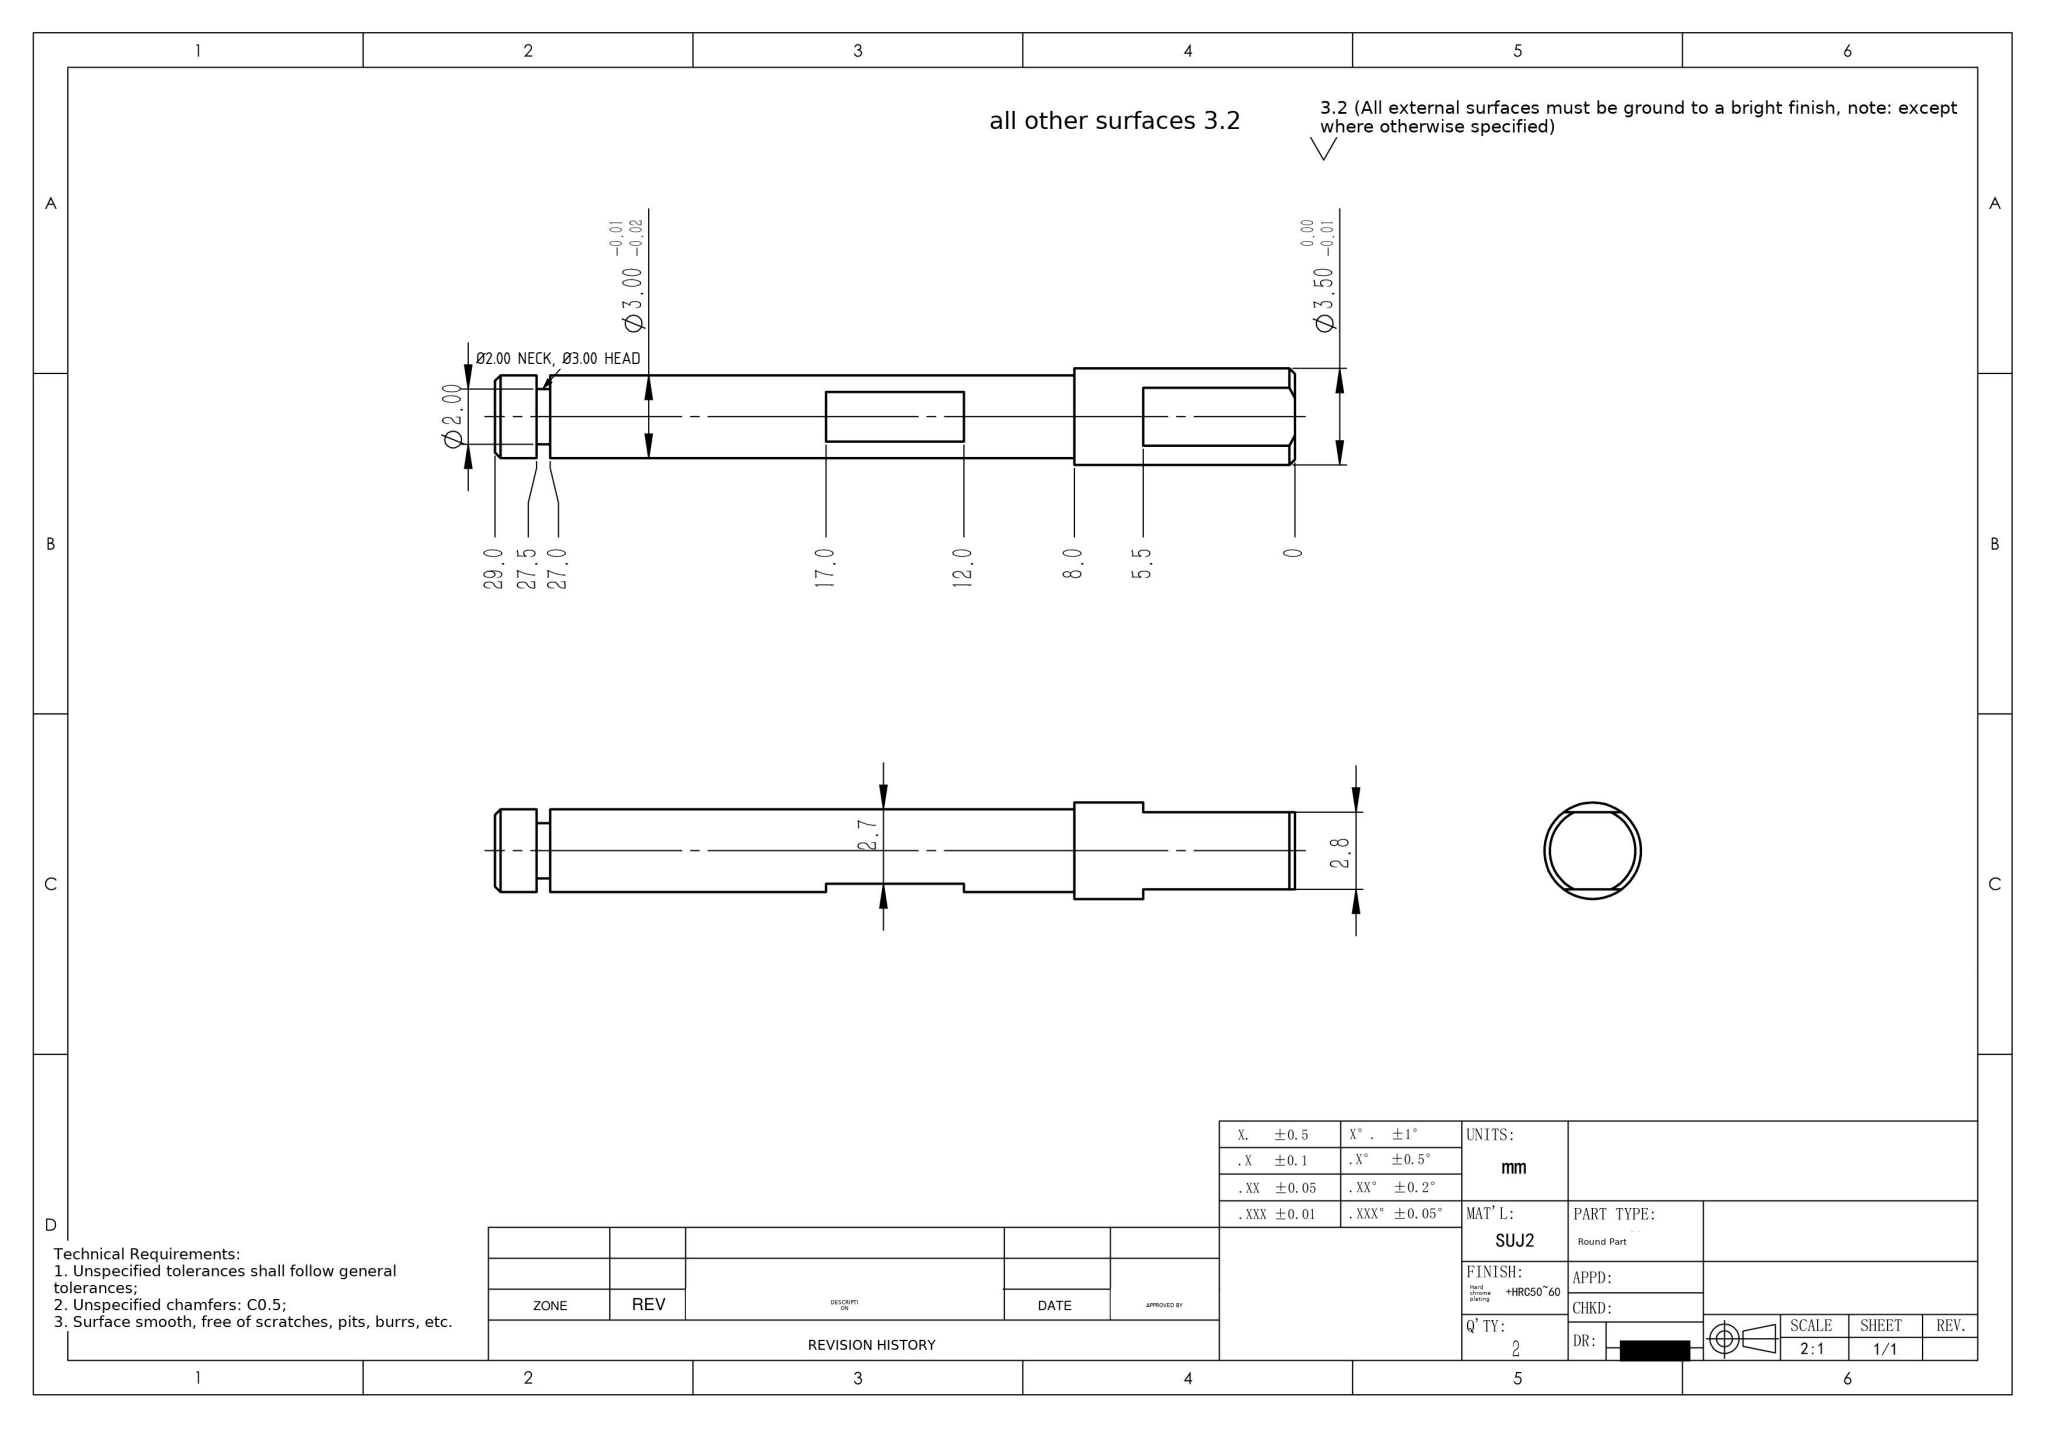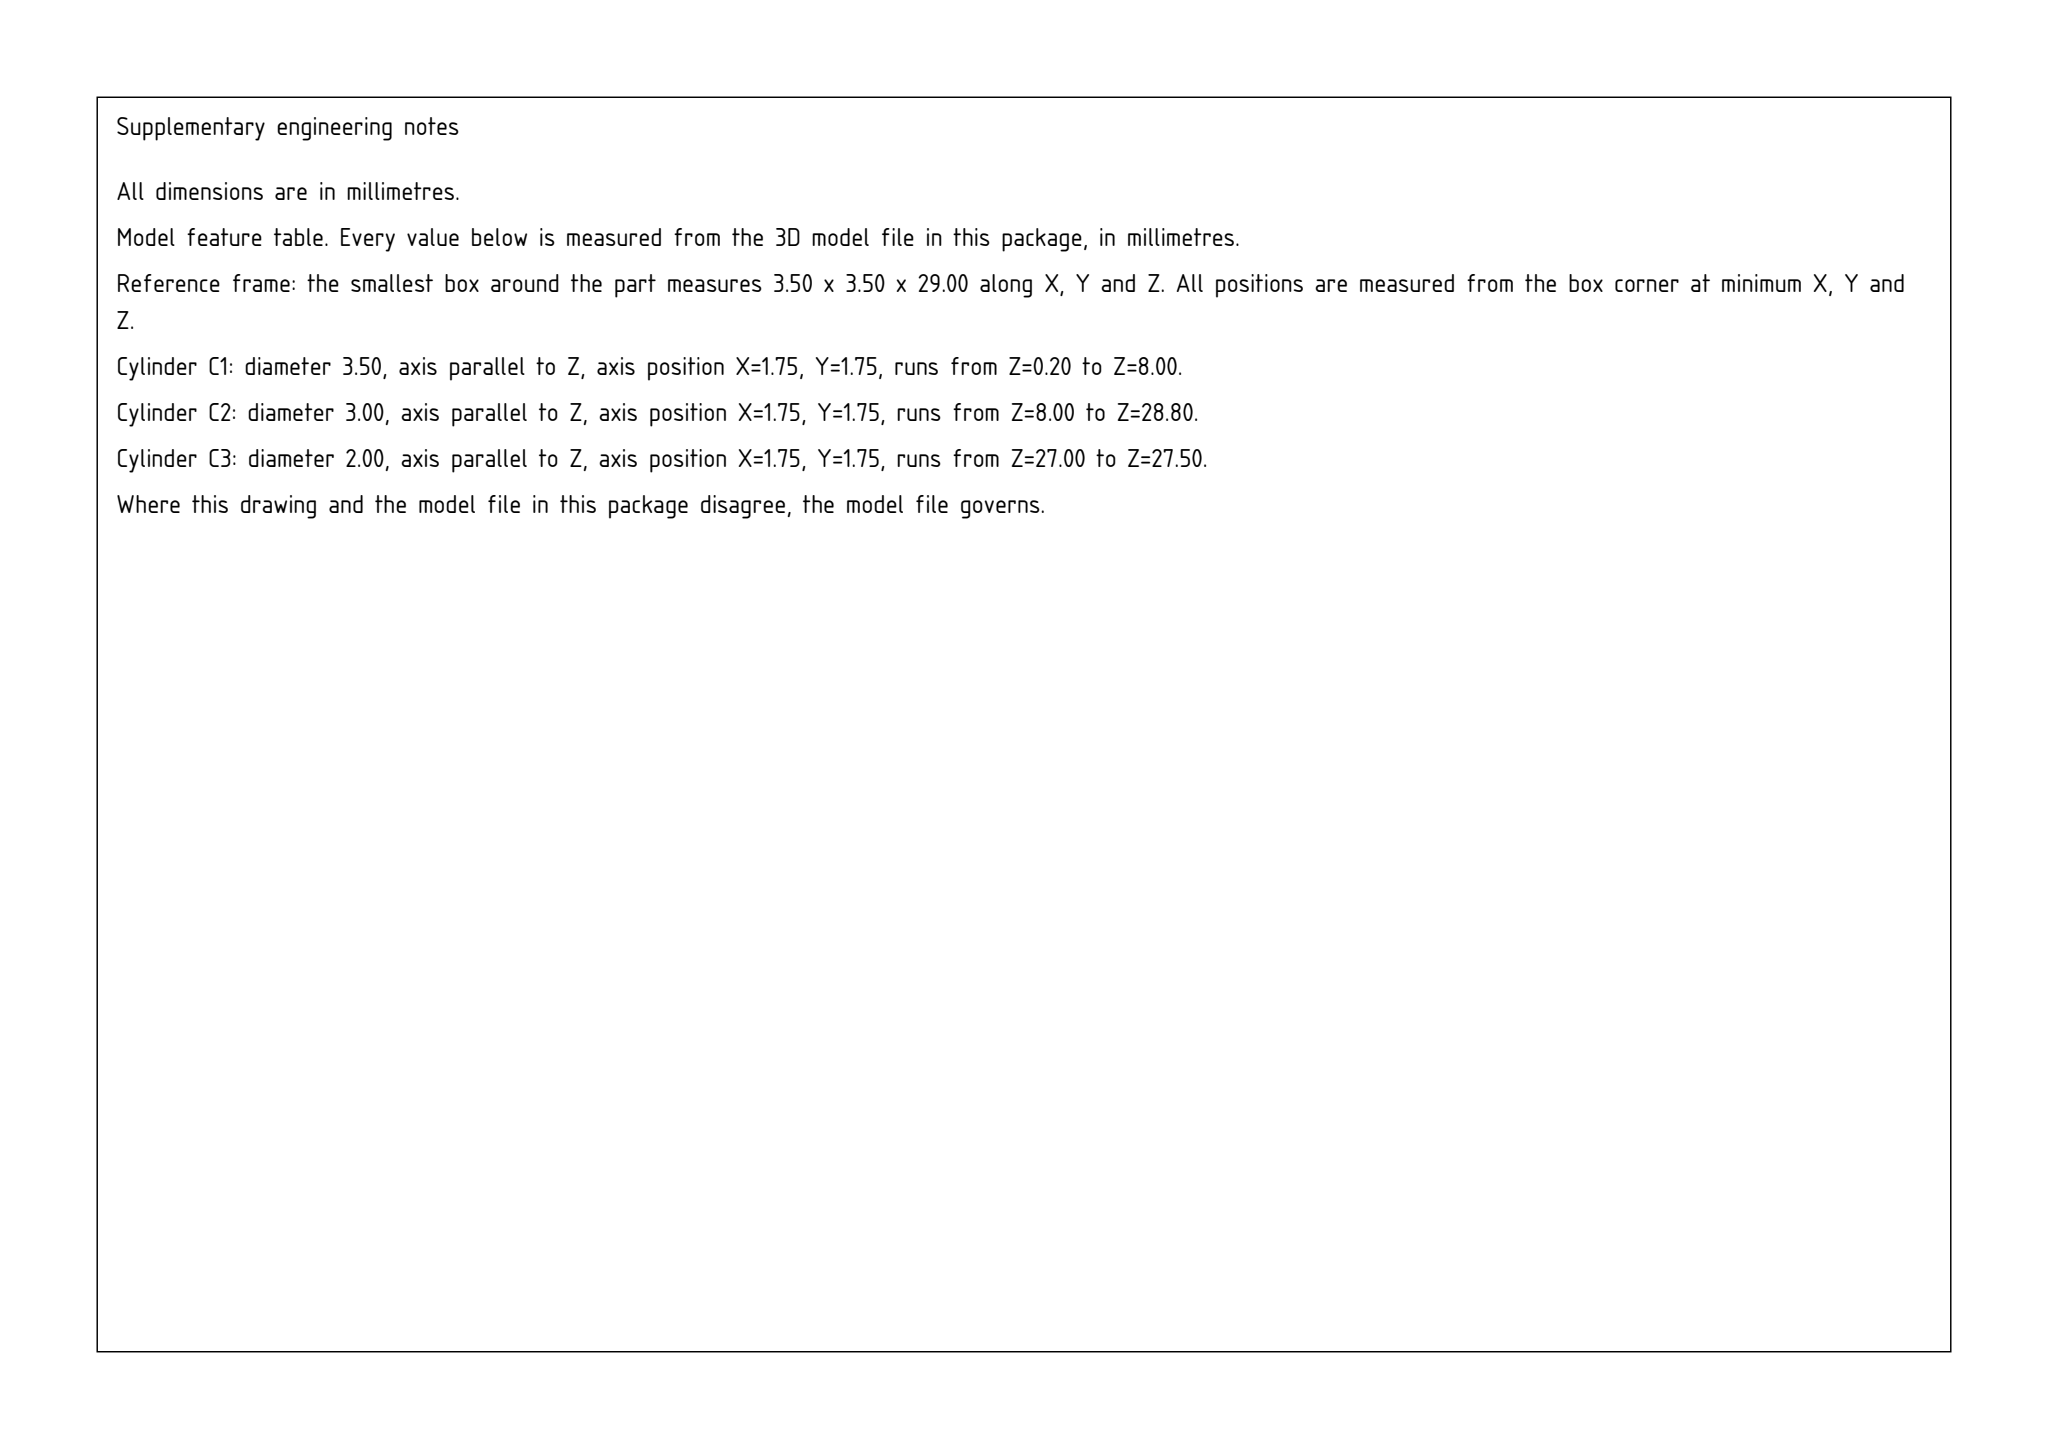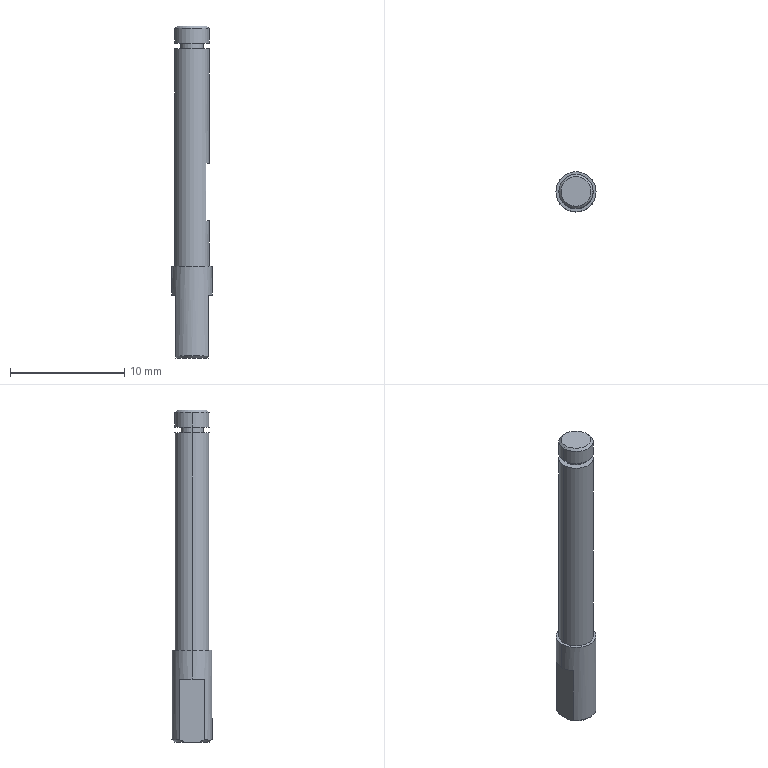Part | SolidWorks | mm | material SUJ2 | 1 solid | 24 faces | box 3.5 x 3.5 x 29 mm | volume 216 mm3 | plane 12 | cylinder 8 | cone 4 | commonest cylinder face diameters 3 x4 2 x2 3.5 x2
Drawing notes:
HEAD Ø3.00 FROM 27.5 TO 29.0; NECK Ø2.00 FROM 27.0 TO 27.5 | from the solid: cyl dia 3.0 z 27.5-28.8 (+90° cone to 29.0); cyl dia 2.0 z 27.0-27.5; both on axis x=y=1.8
build123d program:
from build123d import *

# Parameters (mm, degrees)
SKETCH1_R           = 1.75
BOSS_EXTRUDE1_DEPTH = 29
SKETCH2_OUTSIDE_W   = 11.384
SKETCH2_OUTSIDE_H   = 11.384
SKETCH2_OUTSIDE_R   = 1.5
CUT_EXTRUDE1_DEPTH  = 21
CUT_EXTRUDE2_START  = -1.5
SKETCH3_OUTSIDE_W   = 11.384
SKETCH3_OUTSIDE_H   = 11.384
SKETCH3_OUTSIDE_R   = 1
CUT_EXTRUDE2_DEPTH  = 0.5
CUT_EXTRUDE3_START  = -17
SKETCH4_W           = 2
SKETCH4_H           = 3
CUT_EXTRUDE3_DEPTH  = 5
SKETCH5_OUTSIDE_W   = 11.384
SKETCH5_OUTSIDE_H   = 11.384
SKETCH5_OUTSIDE_W_2 = 2.8
SKETCH5_OUTSIDE_H_2 = 5
CUT_EXTRUDE4_DEPTH  = 5.5
CHAMFER1_SIZE       = 0.2


with BuildPart() as part:
    # Sketch1 → Boss-Extrude1 (new body)
    with BuildSketch(Plane.XY):
        with Locations(Location((0, 0, 0), (0, 0, 180))):
            Circle(SKETCH1_R)
    extrude(amount=BOSS_EXTRUDE1_DEPTH)

    # Sketch2 outside → Cut-Extrude1 (cut)
    with BuildSketch(Plane.XY.offset(29)):
        Rectangle(SKETCH2_OUTSIDE_W, SKETCH2_OUTSIDE_H)
        Circle(SKETCH2_OUTSIDE_R, mode=Mode.SUBTRACT)
    extrude(amount=-CUT_EXTRUDE1_DEPTH, mode=Mode.SUBTRACT)

    # Sketch3 outside → Cut-Extrude2 (cut)
    with BuildSketch(Plane.XY.offset(29).offset(CUT_EXTRUDE2_START)):
        Rectangle(SKETCH3_OUTSIDE_W, SKETCH3_OUTSIDE_H)
        Circle(SKETCH3_OUTSIDE_R, mode=Mode.SUBTRACT)
    extrude(amount=-CUT_EXTRUDE2_DEPTH, mode=Mode.SUBTRACT)

    # Sketch4 → Cut-Extrude3 (cut)
    with BuildSketch(Plane.XY.offset(29).offset(CUT_EXTRUDE3_START)):
        with Locations((2.2, 0)):
            Rectangle(SKETCH4_W, SKETCH4_H)
    extrude(amount=CUT_EXTRUDE3_DEPTH, mode=Mode.SUBTRACT)

    # Sketch5 outside → Cut-Extrude4 (cut)
    with BuildSketch(Plane(origin=(0, 0, 0), x_dir=(-1, 0, 0), z_dir=(0, 0, -1))):
        Rectangle(SKETCH5_OUTSIDE_W, SKETCH5_OUTSIDE_H)
        Rectangle(SKETCH5_OUTSIDE_W_2, SKETCH5_OUTSIDE_H_2, mode=Mode.SUBTRACT)
    extrude(amount=-CUT_EXTRUDE4_DEPTH, mode=Mode.SUBTRACT)

    # Chamfer1
    chamfer1_edges = [part.edges().sort_by_distance(p)[0] for p in [
        (-1.5, 0, 29),
        (0, 1.75, 0),
        (0, -1.75, 0),
    ]]
    chamfer(chamfer1_edges, length=CHAMFER1_SIZE)


solid = part.part
STEP:
#1=CARTESIAN_POINT('',(1.3,0.,29.));
#2=VERTEX_POINT('',#1);
#3=CARTESIAN_POINT('',(-1.3,0.,29.));
#4=VERTEX_POINT('',#3);
#5=CARTESIAN_POINT('',(0.,0.,29.));
#6=DIRECTION('',(0.,0.,1.));
#7=DIRECTION('',(1.,0.,0.));
#8=AXIS2_PLACEMENT_3D('',#5,#6,#7);
#9=CIRCLE('',#8,1.3);
#10=EDGE_CURVE('',#2,#4,#9,.T.);
#11=ORIENTED_EDGE('',*,*,#10,.F.);
#12=CARTESIAN_POINT('',(1.5,0.,28.8));
#13=VERTEX_POINT('',#12);
#14=CARTESIAN_POINT('',(1.3,0.,29.));
#15=DIRECTION('',(0.7071,0.,-0.7071));
#16=VECTOR('',#15,1000.);
#17=LINE('',#14,#16);
#18=EDGE_CURVE('',#2,#13,#17,.T.);
#19=ORIENTED_EDGE('',*,*,#18,.T.);
#20=CARTESIAN_POINT('',(-1.5,0.,28.8));
#21=VERTEX_POINT('',#20);
#22=CARTESIAN_POINT('',(0.,0.,28.8));
#23=DIRECTION('',(0.,0.,-1.));
#24=DIRECTION('',(1.,0.,0.));
#25=AXIS2_PLACEMENT_3D('',#22,#23,#24);
#26=CIRCLE('',#25,1.5);
#27=EDGE_CURVE('',#21,#13,#26,.T.);
#28=ORIENTED_EDGE('',*,*,#27,.F.);
#29=CARTESIAN_POINT('',(-1.3,0.,29.));
#30=DIRECTION('',(-0.7071,0.,-0.7071));
#31=VECTOR('',#30,1000.);
#32=LINE('',#29,#31);
#33=EDGE_CURVE('',#4,#21,#32,.T.);
#34=ORIENTED_EDGE('',*,*,#33,.F.);
#35=EDGE_LOOP('',(#11,#19,#28,#34));
#36=FACE_OUTER_BOUND('',#35,.T.);
#37=CARTESIAN_POINT('',(0.,0.,29.));
#38=DIRECTION('',(0.,0.,-1.));
#39=DIRECTION('',(-1.,0.,0.));
#40=AXIS2_PLACEMENT_3D('',#37,#38,#39);
#41=CONICAL_SURFACE('',#40,1.3,0.7854);
#42=ADVANCED_FACE('',(#36),#41,.T.);
#43=CARTESIAN_POINT('',(-1.5,0.,27.5));
#44=VERTEX_POINT('',#43);
#45=CARTESIAN_POINT('',(1.5,0.,27.5));
#46=VERTEX_POINT('',#45);
#47=CARTESIAN_POINT('',(0.,0.,27.5));
#48=DIRECTION('',(0.,0.,-1.));
#49=DIRECTION('',(1.,0.,0.));
#50=AXIS2_PLACEMENT_3D('',#47,#48,#49);
#51=CIRCLE('',#50,1.5);
#52=EDGE_CURVE('',#44,#46,#51,.T.);
#53=ORIENTED_EDGE('',*,*,#52,.F.);
#54=CARTESIAN_POINT('',(-1.5,0.,8.));
#55=DIRECTION('',(0.,0.,1.));
#56=VECTOR('',#55,1000.);
#57=LINE('',#54,#56);
#58=EDGE_CURVE('',#44,#21,#57,.T.);
#59=ORIENTED_EDGE('',*,*,#58,.T.);
#60=ORIENTED_EDGE('',*,*,#27,.T.);
#61=CARTESIAN_POINT('',(1.5,0.,8.));
#62=DIRECTION('',(0.,0.,1.));
#63=VECTOR('',#62,1000.);
#64=LINE('',#61,#63);
#65=EDGE_CURVE('',#46,#13,#64,.T.);
#66=ORIENTED_EDGE('',*,*,#65,.F.);
#67=EDGE_LOOP('',(#53,#59,#60,#66));
#68=FACE_OUTER_BOUND('',#67,.T.);
#69=CARTESIAN_POINT('',(0.,0.,8.));
#70=DIRECTION('',(0.,0.,1.));
#71=DIRECTION('',(1.,0.,0.));
#72=AXIS2_PLACEMENT_3D('',#69,#70,#71);
#73=CYLINDRICAL_SURFACE('',#72,1.5);
#74=ADVANCED_FACE('',(#68),#73,.T.);
#75=CARTESIAN_POINT('',(1.,0.,27.));
#76=VERTEX_POINT('',#75);
#77=CARTESIAN_POINT('',(-1.,0.,27.));
#78=VERTEX_POINT('',#77);
#79=CARTESIAN_POINT('',(0.,0.,27.));
#80=DIRECTION('',(0.,0.,1.));
#81=DIRECTION('',(1.,0.,0.));
#82=AXIS2_PLACEMENT_3D('',#79,#80,#81);
#83=CIRCLE('',#82,1.);
#84=EDGE_CURVE('',#76,#78,#83,.T.);
#85=ORIENTED_EDGE('',*,*,#84,.T.);
#86=CARTESIAN_POINT('',(-1.,0.,27.5));
#87=VERTEX_POINT('',#86);
#88=CARTESIAN_POINT('',(-1.,0.,27.));
#89=DIRECTION('',(0.,0.,1.));
#90=VECTOR('',#89,1000.);
#91=LINE('',#88,#90);
#92=EDGE_CURVE('',#78,#87,#91,.T.);
#93=ORIENTED_EDGE('',*,*,#92,.T.);
#94=CARTESIAN_POINT('',(1.,0.,27.5));
#95=VERTEX_POINT('',#94);
#96=CARTESIAN_POINT('',(0.,0.,27.5));
#97=DIRECTION('',(0.,0.,1.));
#98=DIRECTION('',(1.,0.,0.));
#99=AXIS2_PLACEMENT_3D('',#96,#97,#98);
#100=CIRCLE('',#99,1.);
#101=EDGE_CURVE('',#95,#87,#100,.T.);
#102=ORIENTED_EDGE('',*,*,#101,.F.);
#103=CARTESIAN_POINT('',(1.,0.,27.));
#104=DIRECTION('',(0.,0.,1.));
#105=VECTOR('',#104,1000.);
#106=LINE('',#103,#105);
#107=EDGE_CURVE('',#76,#95,#106,.T.);
#108=ORIENTED_EDGE('',*,*,#107,.F.);
#109=EDGE_LOOP('',(#85,#93,#102,#108));
#110=FACE_OUTER_BOUND('',#109,.T.);
#111=CARTESIAN_POINT('',(0.,0.,27.));
#112=DIRECTION('',(0.,0.,1.));
#113=DIRECTION('',(1.,0.,0.));
#114=AXIS2_PLACEMENT_3D('',#111,#112,#113);
#115=CYLINDRICAL_SURFACE('',#114,1.);
#116=ADVANCED_FACE('',(#110),#115,.T.);
#117=CARTESIAN_POINT('',(1.5,0.,8.));
#118=VERTEX_POINT('',#117);
#119=CARTESIAN_POINT('',(-1.5,0.,8.));
#120=VERTEX_POINT('',#119);
#121=CARTESIAN_POINT('',(0.,0.,8.));
#122=DIRECTION('',(0.,0.,1.));
#123=DIRECTION('',(1.,0.,0.));
#124=AXIS2_PLACEMENT_3D('',#121,#122,#123);
#125=CIRCLE('',#124,1.5);
#126=EDGE_CURVE('',#118,#120,#125,.T.);
#127=ORIENTED_EDGE('',*,*,#126,.T.);
#128=CARTESIAN_POINT('',(-1.5,0.,27.));
#129=VERTEX_POINT('',#128);
#130=CARTESIAN_POINT('',(-1.5,0.,8.));
#131=DIRECTION('',(0.,0.,1.));
#132=VECTOR('',#131,1000.);
#133=LINE('',#130,#132);
#134=EDGE_CURVE('',#120,#129,#133,.T.);
#135=ORIENTED_EDGE('',*,*,#134,.T.);
#136=CARTESIAN_POINT('',(1.5,0.,27.));
#137=VERTEX_POINT('',#136);
#138=CARTESIAN_POINT('',(0.,0.,27.));
#139=DIRECTION('',(0.,0.,-1.));
#140=DIRECTION('',(1.,0.,0.));
#141=AXIS2_PLACEMENT_3D('',#138,#139,#140);
#142=CIRCLE('',#141,1.5);
#143=EDGE_CURVE('',#129,#137,#142,.T.);
#144=ORIENTED_EDGE('',*,*,#143,.T.);
#145=CARTESIAN_POINT('',(1.5,0.,17.));
#146=VERTEX_POINT('',#145);
#147=CARTESIAN_POINT('',(1.5,0.,8.));
#148=DIRECTION('',(0.,0.,1.));
#149=VECTOR('',#148,1000.);
#150=LINE('',#147,#149);
#151=EDGE_CURVE('',#146,#137,#150,.T.);
#152=ORIENTED_EDGE('',*,*,#151,.F.);
#153=CARTESIAN_POINT('',(1.2,0.9,17.));
#154=VERTEX_POINT('',#153);
#155=CARTESIAN_POINT('',(0.,0.,17.));
#156=DIRECTION('',(0.,0.,-1.));
#157=DIRECTION('',(1.,0.,0.));
#158=AXIS2_PLACEMENT_3D('',#155,#156,#157);
#159=CIRCLE('',#158,1.5);
#160=EDGE_CURVE('',#154,#146,#159,.T.);
#161=ORIENTED_EDGE('',*,*,#160,.F.);
#162=CARTESIAN_POINT('',(1.2,0.9,12.));
#163=VERTEX_POINT('',#162);
#164=CARTESIAN_POINT('',(1.2,0.9,8.));
#165=DIRECTION('',(0.,0.,-1.));
#166=VECTOR('',#165,1000.);
#167=LINE('',#164,#166);
#168=EDGE_CURVE('',#154,#163,#167,.T.);
#169=ORIENTED_EDGE('',*,*,#168,.T.);
#170=CARTESIAN_POINT('',(1.5,0.,12.));
#171=VERTEX_POINT('',#170);
#172=CARTESIAN_POINT('',(0.,0.,12.));
#173=DIRECTION('',(0.,0.,-1.));
#174=DIRECTION('',(1.,0.,0.));
#175=AXIS2_PLACEMENT_3D('',#172,#173,#174);
#176=CIRCLE('',#175,1.5);
#177=EDGE_CURVE('',#163,#171,#176,.T.);
#178=ORIENTED_EDGE('',*,*,#177,.T.);
#179=CARTESIAN_POINT('',(1.5,0.,8.));
#180=DIRECTION('',(0.,0.,1.));
#181=VECTOR('',#180,1000.);
#182=LINE('',#179,#181);
#183=EDGE_CURVE('',#118,#171,#182,.T.);
#184=ORIENTED_EDGE('',*,*,#183,.F.);
#185=EDGE_LOOP('',(#127,#135,#144,#152,#161,#169,#178,#184));
#186=FACE_OUTER_BOUND('',#185,.T.);
#187=CARTESIAN_POINT('',(0.,0.,8.));
#188=DIRECTION('',(0.,0.,1.));
#189=DIRECTION('',(1.,0.,0.));
#190=AXIS2_PLACEMENT_3D('',#187,#188,#189);
#191=CYLINDRICAL_SURFACE('',#190,1.5);
#192=ADVANCED_FACE('',(#186),#191,.T.);
#193=CARTESIAN_POINT('',(1.75,0.,8.));
#194=VERTEX_POINT('',#193);
#195=CARTESIAN_POINT('',(-1.75,0.,8.));
#196=VERTEX_POINT('',#195);
#197=CARTESIAN_POINT('',(0.,0.,8.));
#198=DIRECTION('',(0.,0.,1.));
#199=DIRECTION('',(1.,0.,0.));
#200=AXIS2_PLACEMENT_3D('',#197,#198,#199);
#201=CIRCLE('',#200,1.75);
#202=EDGE_CURVE('',#194,#196,#201,.T.);
#203=ORIENTED_EDGE('',*,*,#202,.F.);
#204=CARTESIAN_POINT('',(1.75,0.,5.5));
#205=VERTEX_POINT('',#204);
#206=CARTESIAN_POINT('',(1.75,0.,29.));
#207=DIRECTION('',(0.,0.,-1.));
#208=VECTOR('',#207,1000.);
#209=LINE('',#206,#208);
#210=EDGE_CURVE('',#194,#205,#209,.T.);
#211=ORIENTED_EDGE('',*,*,#210,.T.);
#212=CARTESIAN_POINT('',(1.4,1.05,5.5));
#213=VERTEX_POINT('',#212);
#214=CARTESIAN_POINT('',(0.,0.,5.5));
#215=DIRECTION('',(0.,0.,-1.));
#216=DIRECTION('',(-1.,0.,0.));
#217=AXIS2_PLACEMENT_3D('',#214,#215,#216);
#218=CIRCLE('',#217,1.75);
#219=EDGE_CURVE('',#213,#205,#218,.T.);
#220=ORIENTED_EDGE('',*,*,#219,.F.);
#221=CARTESIAN_POINT('',(1.4,1.05,0.2));
#222=VERTEX_POINT('',#221);
#223=CARTESIAN_POINT('',(1.4,1.05,29.));
#224=DIRECTION('',(0.,0.,1.));
#225=VECTOR('',#224,1000.);
#226=LINE('',#223,#225);
#227=EDGE_CURVE('',#222,#213,#226,.T.);
#228=ORIENTED_EDGE('',*,*,#227,.F.);
#229=CARTESIAN_POINT('',(-1.4,1.05,0.2));
#230=VERTEX_POINT('',#229);
#231=CARTESIAN_POINT('',(0.,0.,0.2));
#232=DIRECTION('',(0.,0.,1.));
#233=DIRECTION('',(1.,0.,0.));
#234=AXIS2_PLACEMENT_3D('',#231,#232,#233);
#235=CIRCLE('',#234,1.75);
#236=EDGE_CURVE('',#222,#230,#235,.T.);
#237=ORIENTED_EDGE('',*,*,#236,.T.);
#238=CARTESIAN_POINT('',(-1.4,1.05,5.5));
#239=VERTEX_POINT('',#238);
#240=CARTESIAN_POINT('',(-1.4,1.05,29.));
#241=DIRECTION('',(0.,0.,-1.));
#242=VECTOR('',#241,1000.);
#243=LINE('',#240,#242);
#244=EDGE_CURVE('',#239,#230,#243,.T.);
#245=ORIENTED_EDGE('',*,*,#244,.F.);
#246=CARTESIAN_POINT('',(-1.75,0.,5.5));
#247=VERTEX_POINT('',#246);
#248=CARTESIAN_POINT('',(0.,0.,5.5));
#249=DIRECTION('',(0.,0.,-1.));
#250=DIRECTION('',(-1.,0.,0.));
#251=AXIS2_PLACEMENT_3D('',#248,#249,#250);
#252=CIRCLE('',#251,1.75);
#253=EDGE_CURVE('',#247,#239,#252,.T.);
#254=ORIENTED_EDGE('',*,*,#253,.F.);
#255=CARTESIAN_POINT('',(-1.75,0.,29.));
#256=DIRECTION('',(0.,0.,-1.));
#257=VECTOR('',#256,1000.);
#258=LINE('',#255,#257);
#259=EDGE_CURVE('',#196,#247,#258,.T.);
#260=ORIENTED_EDGE('',*,*,#259,.F.);
#261=EDGE_LOOP('',(#203,#211,#220,#228,#237,#245,#254,#260));
#262=FACE_OUTER_BOUND('',#261,.T.);
#263=CARTESIAN_POINT('',(0.,0.,29.));
#264=DIRECTION('',(0.,0.,-1.));
#265=DIRECTION('',(-1.,0.,0.));
#266=AXIS2_PLACEMENT_3D('',#263,#264,#265);
#267=CYLINDRICAL_SURFACE('',#266,1.75);
#268=ADVANCED_FACE('',(#262),#267,.T.);
#269=ORIENTED_EDGE('',*,*,#210,.F.);
#270=CARTESIAN_POINT('',(0.,0.,8.));
#271=DIRECTION('',(0.,0.,1.));
#272=DIRECTION('',(1.,0.,0.));
#273=AXIS2_PLACEMENT_3D('',#270,#271,#272);
#274=CIRCLE('',#273,1.75);
#275=EDGE_CURVE('',#196,#194,#274,.T.);
#276=ORIENTED_EDGE('',*,*,#275,.F.);
#277=ORIENTED_EDGE('',*,*,#259,.T.);
#278=CARTESIAN_POINT('',(-1.4,-1.05,5.5));
#279=VERTEX_POINT('',#278);
#280=CARTESIAN_POINT('',(0.,0.,5.5));
#281=DIRECTION('',(0.,0.,-1.));
#282=DIRECTION('',(-1.,0.,0.));
#283=AXIS2_PLACEMENT_3D('',#280,#281,#282);
#284=CIRCLE('',#283,1.75);
#285=EDGE_CURVE('',#279,#247,#284,.T.);
#286=ORIENTED_EDGE('',*,*,#285,.F.);
#287=CARTESIAN_POINT('',(-1.4,-1.05,0.2));
#288=VERTEX_POINT('',#287);
#289=CARTESIAN_POINT('',(-1.4,-1.05,29.));
#290=DIRECTION('',(0.,0.,1.));
#291=VECTOR('',#290,1000.);
#292=LINE('',#289,#291);
#293=EDGE_CURVE('',#288,#279,#292,.T.);
#294=ORIENTED_EDGE('',*,*,#293,.F.);
#295=CARTESIAN_POINT('',(1.4,-1.05,0.2));
#296=VERTEX_POINT('',#295);
#297=CARTESIAN_POINT('',(0.,0.,0.2));
#298=DIRECTION('',(0.,0.,1.));
#299=DIRECTION('',(1.,0.,0.));
#300=AXIS2_PLACEMENT_3D('',#297,#298,#299);
#301=CIRCLE('',#300,1.75);
#302=EDGE_CURVE('',#288,#296,#301,.T.);
#303=ORIENTED_EDGE('',*,*,#302,.T.);
#304=CARTESIAN_POINT('',(1.4,-1.05,5.5));
#305=VERTEX_POINT('',#304);
#306=CARTESIAN_POINT('',(1.4,-1.05,29.));
#307=DIRECTION('',(0.,0.,-1.));
#308=VECTOR('',#307,1000.);
#309=LINE('',#306,#308);
#310=EDGE_CURVE('',#305,#296,#309,.T.);
#311=ORIENTED_EDGE('',*,*,#310,.F.);
#312=CARTESIAN_POINT('',(0.,0.,5.5));
#313=DIRECTION('',(0.,0.,-1.));
#314=DIRECTION('',(-1.,0.,0.));
#315=AXIS2_PLACEMENT_3D('',#312,#313,#314);
#316=CIRCLE('',#315,1.75);
#317=EDGE_CURVE('',#205,#305,#316,.T.);
#318=ORIENTED_EDGE('',*,*,#317,.F.);
#319=EDGE_LOOP('',(#269,#276,#277,#286,#294,#303,#311,#318));
#320=FACE_OUTER_BOUND('',#319,.T.);
#321=CARTESIAN_POINT('',(0.,0.,29.));
#322=DIRECTION('',(0.,0.,-1.));
#323=DIRECTION('',(-1.,0.,0.));
#324=AXIS2_PLACEMENT_3D('',#321,#322,#323);
#325=CYLINDRICAL_SURFACE('',#324,1.75);
#326=ADVANCED_FACE('',(#320),#325,.T.);
#327=CARTESIAN_POINT('',(1.4,-0.6652,0.));
#328=VERTEX_POINT('',#327);
#329=CARTESIAN_POINT('',(1.4,0.6652,0.));
#330=VERTEX_POINT('',#329);
#331=CARTESIAN_POINT('',(1.4,0.,0.));
#332=DIRECTION('',(0.,1.,0.));
#333=VECTOR('',#332,1000.);
#334=LINE('',#331,#333);
#335=EDGE_CURVE('',#328,#330,#334,.T.);
#336=ORIENTED_EDGE('',*,*,#335,.F.);
#337=CARTESIAN_POINT('',(-1.4,-0.6652,0.));
#338=VERTEX_POINT('',#337);
#339=CARTESIAN_POINT('',(0.,0.,0.));
#340=DIRECTION('',(0.,0.,-1.));
#341=DIRECTION('',(1.,0.,0.));
#342=AXIS2_PLACEMENT_3D('',#339,#340,#341);
#343=CIRCLE('',#342,1.55);
#344=EDGE_CURVE('',#328,#338,#343,.T.);
#345=ORIENTED_EDGE('',*,*,#344,.T.);
#346=CARTESIAN_POINT('',(-1.4,0.6652,0.));
#347=VERTEX_POINT('',#346);
#348=CARTESIAN_POINT('',(-1.4,0.,0.));
#349=DIRECTION('',(0.,-1.,0.));
#350=VECTOR('',#349,1000.);
#351=LINE('',#348,#350);
#352=EDGE_CURVE('',#347,#338,#351,.T.);
#353=ORIENTED_EDGE('',*,*,#352,.F.);
#354=CARTESIAN_POINT('',(0.,0.,0.));
#355=DIRECTION('',(0.,0.,-1.));
#356=DIRECTION('',(1.,0.,0.));
#357=AXIS2_PLACEMENT_3D('',#354,#355,#356);
#358=CIRCLE('',#357,1.55);
#359=EDGE_CURVE('',#347,#330,#358,.T.);
#360=ORIENTED_EDGE('',*,*,#359,.T.);
#361=EDGE_LOOP('',(#336,#345,#353,#360));
#362=FACE_OUTER_BOUND('',#361,.T.);
#363=CARTESIAN_POINT('',(0.,0.,0.));
#364=DIRECTION('',(0.,0.,1.));
#365=DIRECTION('',(1.,0.,0.));
#366=AXIS2_PLACEMENT_3D('',#363,#364,#365);
#367=PLANE('',#366);
#368=ADVANCED_FACE('',(#362),#367,.F.);
#369=ORIENTED_EDGE('',*,*,#134,.F.);
#370=CARTESIAN_POINT('',(0.,0.,8.));
#371=DIRECTION('',(0.,0.,1.));
#372=DIRECTION('',(1.,0.,0.));
#373=AXIS2_PLACEMENT_3D('',#370,#371,#372);
#374=CIRCLE('',#373,1.5);
#375=EDGE_CURVE('',#120,#118,#374,.T.);
#376=ORIENTED_EDGE('',*,*,#375,.T.);
#377=ORIENTED_EDGE('',*,*,#183,.T.);
#378=CARTESIAN_POINT('',(1.2,-0.9,12.));
#379=VERTEX_POINT('',#378);
#380=CARTESIAN_POINT('',(0.,0.,12.));
#381=DIRECTION('',(0.,0.,-1.));
#382=DIRECTION('',(1.,0.,0.));
#383=AXIS2_PLACEMENT_3D('',#380,#381,#382);
#384=CIRCLE('',#383,1.5);
#385=EDGE_CURVE('',#171,#379,#384,.T.);
#386=ORIENTED_EDGE('',*,*,#385,.T.);
#387=CARTESIAN_POINT('',(1.2,-0.9,17.));
#388=VERTEX_POINT('',#387);
#389=CARTESIAN_POINT('',(1.2,-0.9,8.));
#390=DIRECTION('',(0.,0.,1.));
#391=VECTOR('',#390,1000.);
#392=LINE('',#389,#391);
#393=EDGE_CURVE('',#379,#388,#392,.T.);
#394=ORIENTED_EDGE('',*,*,#393,.T.);
#395=CARTESIAN_POINT('',(0.,0.,17.));
#396=DIRECTION('',(0.,0.,-1.));
#397=DIRECTION('',(1.,0.,0.));
#398=AXIS2_PLACEMENT_3D('',#395,#396,#397);
#399=CIRCLE('',#398,1.5);
#400=EDGE_CURVE('',#146,#388,#399,.T.);
#401=ORIENTED_EDGE('',*,*,#400,.F.);
#402=ORIENTED_EDGE('',*,*,#151,.T.);
#403=CARTESIAN_POINT('',(0.,0.,27.));
#404=DIRECTION('',(0.,0.,-1.));
#405=DIRECTION('',(1.,0.,0.));
#406=AXIS2_PLACEMENT_3D('',#403,#404,#405);
#407=CIRCLE('',#406,1.5);
#408=EDGE_CURVE('',#137,#129,#407,.T.);
#409=ORIENTED_EDGE('',*,*,#408,.T.);
#410=EDGE_LOOP('',(#369,#376,#377,#386,#394,#401,#402,#409));
#411=FACE_OUTER_BOUND('',#410,.T.);
#412=CARTESIAN_POINT('',(0.,0.,8.));
#413=DIRECTION('',(0.,0.,1.));
#414=DIRECTION('',(1.,0.,0.));
#415=AXIS2_PLACEMENT_3D('',#412,#413,#414);
#416=CYLINDRICAL_SURFACE('',#415,1.5);
#417=ADVANCED_FACE('',(#411),#416,.T.);
#418=ORIENTED_EDGE('',*,*,#126,.F.);
#419=ORIENTED_EDGE('',*,*,#375,.F.);
#420=EDGE_LOOP('',(#418,#419));
#421=FACE_BOUND('',#420,.T.);
#422=ORIENTED_EDGE('',*,*,#275,.T.);
#423=ORIENTED_EDGE('',*,*,#202,.T.);
#424=EDGE_LOOP('',(#422,#423));
#425=FACE_OUTER_BOUND('',#424,.T.);
#426=CARTESIAN_POINT('',(0.,0.,8.));
#427=DIRECTION('',(0.,0.,1.));
#428=DIRECTION('',(1.,0.,0.));
#429=AXIS2_PLACEMENT_3D('',#426,#427,#428);
#430=PLANE('',#429);
#431=ADVANCED_FACE('',(#421,#425),#430,.T.);
#432=ORIENTED_EDGE('',*,*,#408,.F.);
#433=ORIENTED_EDGE('',*,*,#143,.F.);
#434=EDGE_LOOP('',(#432,#433));
#435=FACE_OUTER_BOUND('',#434,.T.);
#436=ORIENTED_EDGE('',*,*,#84,.F.);
#437=CARTESIAN_POINT('',(0.,0.,27.));
#438=DIRECTION('',(0.,0.,1.));
#439=DIRECTION('',(1.,0.,0.));
#440=AXIS2_PLACEMENT_3D('',#437,#438,#439);
#441=CIRCLE('',#440,1.);
#442=EDGE_CURVE('',#78,#76,#441,.T.);
#443=ORIENTED_EDGE('',*,*,#442,.F.);
#444=EDGE_LOOP('',(#436,#443));
#445=FACE_BOUND('',#444,.T.);
#446=CARTESIAN_POINT('',(0.,0.,27.));
#447=DIRECTION('',(0.,0.,1.));
#448=DIRECTION('',(1.,0.,0.));
#449=AXIS2_PLACEMENT_3D('',#446,#447,#448);
#450=PLANE('',#449);
#451=ADVANCED_FACE('',(#435,#445),#450,.T.);
#452=CARTESIAN_POINT('',(0.,0.,27.5));
#453=DIRECTION('',(0.,0.,-1.));
#454=DIRECTION('',(1.,0.,0.));
#455=AXIS2_PLACEMENT_3D('',#452,#453,#454);
#456=CIRCLE('',#455,1.5);
#457=EDGE_CURVE('',#46,#44,#456,.T.);
#458=ORIENTED_EDGE('',*,*,#457,.T.);
#459=ORIENTED_EDGE('',*,*,#52,.T.);
#460=EDGE_LOOP('',(#458,#459));
#461=FACE_OUTER_BOUND('',#460,.T.);
#462=ORIENTED_EDGE('',*,*,#101,.T.);
#463=CARTESIAN_POINT('',(0.,0.,27.5));
#464=DIRECTION('',(0.,0.,1.));
#465=DIRECTION('',(1.,0.,0.));
#466=AXIS2_PLACEMENT_3D('',#463,#464,#465);
#467=CIRCLE('',#466,1.);
#468=EDGE_CURVE('',#87,#95,#467,.T.);
#469=ORIENTED_EDGE('',*,*,#468,.T.);
#470=EDGE_LOOP('',(#462,#469));
#471=FACE_BOUND('',#470,.T.);
#472=CARTESIAN_POINT('',(0.,0.,27.5));
#473=DIRECTION('',(0.,0.,1.));
#474=DIRECTION('',(1.,0.,0.));
#475=AXIS2_PLACEMENT_3D('',#472,#473,#474);
#476=PLANE('',#475);
#477=ADVANCED_FACE('',(#461,#471),#476,.F.);
#478=ORIENTED_EDGE('',*,*,#92,.F.);
#479=ORIENTED_EDGE('',*,*,#442,.T.);
#480=ORIENTED_EDGE('',*,*,#107,.T.);
#481=ORIENTED_EDGE('',*,*,#468,.F.);
#482=EDGE_LOOP('',(#478,#479,#480,#481));
#483=FACE_OUTER_BOUND('',#482,.T.);
#484=CARTESIAN_POINT('',(0.,0.,27.));
#485=DIRECTION('',(0.,0.,1.));
#486=DIRECTION('',(1.,0.,0.));
#487=AXIS2_PLACEMENT_3D('',#484,#485,#486);
#488=CYLINDRICAL_SURFACE('',#487,1.);
#489=ADVANCED_FACE('',(#483),#488,.T.);
#490=CARTESIAN_POINT('',(0.,0.,29.));
#491=DIRECTION('',(0.,0.,1.));
#492=DIRECTION('',(1.,0.,0.));
#493=AXIS2_PLACEMENT_3D('',#490,#491,#492);
#494=CIRCLE('',#493,1.3);
#495=EDGE_CURVE('',#4,#2,#494,.T.);
#496=ORIENTED_EDGE('',*,*,#495,.T.);
#497=ORIENTED_EDGE('',*,*,#10,.T.);
#498=EDGE_LOOP('',(#496,#497));
#499=FACE_OUTER_BOUND('',#498,.T.);
#500=CARTESIAN_POINT('',(0.,0.,29.));
#501=DIRECTION('',(0.,0.,1.));
#502=DIRECTION('',(1.,0.,0.));
#503=AXIS2_PLACEMENT_3D('',#500,#501,#502);
#504=PLANE('',#503);
#505=ADVANCED_FACE('',(#499),#504,.T.);
#506=ORIENTED_EDGE('',*,*,#58,.F.);
#507=ORIENTED_EDGE('',*,*,#457,.F.);
#508=ORIENTED_EDGE('',*,*,#65,.T.);
#509=CARTESIAN_POINT('',(0.,0.,28.8));
#510=DIRECTION('',(0.,0.,-1.));
#511=DIRECTION('',(1.,0.,0.));
#512=AXIS2_PLACEMENT_3D('',#509,#510,#511);
#513=CIRCLE('',#512,1.5);
#514=EDGE_CURVE('',#13,#21,#513,.T.);
#515=ORIENTED_EDGE('',*,*,#514,.T.);
#516=EDGE_LOOP('',(#506,#507,#508,#515));
#517=FACE_OUTER_BOUND('',#516,.T.);
#518=CARTESIAN_POINT('',(0.,0.,8.));
#519=DIRECTION('',(0.,0.,1.));
#520=DIRECTION('',(1.,0.,0.));
#521=AXIS2_PLACEMENT_3D('',#518,#519,#520);
#522=CYLINDRICAL_SURFACE('',#521,1.5);
#523=ADVANCED_FACE('',(#517),#522,.T.);
#524=CARTESIAN_POINT('',(1.2,1.5,17.));
#525=DIRECTION('',(0.,-1.,0.));
#526=VECTOR('',#525,1000.);
#527=LINE('',#524,#526);
#528=EDGE_CURVE('',#154,#388,#527,.T.);
#529=ORIENTED_EDGE('',*,*,#528,.T.);
#530=ORIENTED_EDGE('',*,*,#393,.F.);
#531=CARTESIAN_POINT('',(1.2,1.5,12.));
#532=DIRECTION('',(0.,-1.,0.));
#533=VECTOR('',#532,1000.);
#534=LINE('',#531,#533);
#535=EDGE_CURVE('',#163,#379,#534,.T.);
#536=ORIENTED_EDGE('',*,*,#535,.F.);
#537=ORIENTED_EDGE('',*,*,#168,.F.);
#538=EDGE_LOOP('',(#529,#530,#536,#537));
#539=FACE_OUTER_BOUND('',#538,.T.);
#540=CARTESIAN_POINT('',(1.2,1.5,17.));
#541=DIRECTION('',(1.,0.,0.));
#542=DIRECTION('',(0.,0.,-1.));
#543=AXIS2_PLACEMENT_3D('',#540,#541,#542);
#544=PLANE('',#543);
#545=ADVANCED_FACE('',(#539),#544,.T.);
#546=ORIENTED_EDGE('',*,*,#160,.T.);
#547=ORIENTED_EDGE('',*,*,#400,.T.);
#548=ORIENTED_EDGE('',*,*,#528,.F.);
#549=EDGE_LOOP('',(#546,#547,#548));
#550=FACE_OUTER_BOUND('',#549,.T.);
#551=CARTESIAN_POINT('',(0.,0.,17.));
#552=DIRECTION('',(0.,0.,1.));
#553=DIRECTION('',(1.,0.,0.));
#554=AXIS2_PLACEMENT_3D('',#551,#552,#553);
#555=PLANE('',#554);
#556=ADVANCED_FACE('',(#550),#555,.F.);
#557=ORIENTED_EDGE('',*,*,#535,.T.);
#558=ORIENTED_EDGE('',*,*,#385,.F.);
#559=ORIENTED_EDGE('',*,*,#177,.F.);
#560=EDGE_LOOP('',(#557,#558,#559));
#561=FACE_OUTER_BOUND('',#560,.T.);
#562=CARTESIAN_POINT('',(0.,0.,12.));
#563=DIRECTION('',(0.,0.,1.));
#564=DIRECTION('',(1.,0.,0.));
#565=AXIS2_PLACEMENT_3D('',#562,#563,#564);
#566=PLANE('',#565);
#567=ADVANCED_FACE('',(#561),#566,.T.);
#568=ORIENTED_EDGE('',*,*,#310,.T.);
#569=CARTESIAN_POINT('',(1.4,-1.05,0.2));
#570=CARTESIAN_POINT('',(1.4,-0.9258,0.1255));
#571=CARTESIAN_POINT('',(1.4,-0.7984,0.05717));
#572=CARTESIAN_POINT('',(1.4,-0.6652,0.));
#573=B_SPLINE_CURVE_WITH_KNOTS('',3,(#569,#570,#571,#572),.UNSPECIFIED.,.F.,.F.,(4,4),(0.,0.0004337),.UNSPECIFIED.);
#574=EDGE_CURVE('',#296,#328,#573,.T.);
#575=ORIENTED_EDGE('',*,*,#574,.T.);
#576=ORIENTED_EDGE('',*,*,#335,.T.);
#577=CARTESIAN_POINT('',(1.4,0.6652,0.));
#578=CARTESIAN_POINT('',(1.4,0.7984,0.05717));
#579=CARTESIAN_POINT('',(1.4,0.9258,0.1255));
#580=CARTESIAN_POINT('',(1.4,1.05,0.2));
#581=B_SPLINE_CURVE_WITH_KNOTS('',3,(#577,#578,#579,#580),.UNSPECIFIED.,.F.,.F.,(4,4),(0.,0.0004337),.UNSPECIFIED.);
#582=EDGE_CURVE('',#330,#222,#581,.T.);
#583=ORIENTED_EDGE('',*,*,#582,.T.);
#584=ORIENTED_EDGE('',*,*,#227,.T.);
#585=CARTESIAN_POINT('',(1.4,-2.5,5.5));
#586=DIRECTION('',(0.,-1.,0.));
#587=VECTOR('',#586,1000.);
#588=LINE('',#585,#587);
#589=EDGE_CURVE('',#213,#305,#588,.T.);
#590=ORIENTED_EDGE('',*,*,#589,.T.);
#591=EDGE_LOOP('',(#568,#575,#576,#583,#584,#590));
#592=FACE_OUTER_BOUND('',#591,.T.);
#593=CARTESIAN_POINT('',(1.4,-2.5,5.5));
#594=DIRECTION('',(1.,0.,0.));
#595=DIRECTION('',(0.,0.,-1.));
#596=AXIS2_PLACEMENT_3D('',#593,#594,#595);
#597=PLANE('',#596);
#598=ADVANCED_FACE('',(#592),#597,.T.);
#599=ORIENTED_EDGE('',*,*,#219,.T.);
#600=ORIENTED_EDGE('',*,*,#317,.T.);
#601=ORIENTED_EDGE('',*,*,#589,.F.);
#602=EDGE_LOOP('',(#599,#600,#601));
#603=FACE_OUTER_BOUND('',#602,.T.);
#604=CARTESIAN_POINT('',(0.,0.,5.5));
#605=DIRECTION('',(0.,0.,-1.));
#606=DIRECTION('',(-1.,0.,0.));
#607=AXIS2_PLACEMENT_3D('',#604,#605,#606);
#608=PLANE('',#607);
#609=ADVANCED_FACE('',(#603),#608,.T.);
#610=ORIENTED_EDGE('',*,*,#285,.T.);
#611=ORIENTED_EDGE('',*,*,#253,.T.);
#612=CARTESIAN_POINT('',(-1.4,-2.5,5.5));
#613=DIRECTION('',(0.,1.,0.));
#614=VECTOR('',#613,1000.);
#615=LINE('',#612,#614);
#616=EDGE_CURVE('',#279,#239,#615,.T.);
#617=ORIENTED_EDGE('',*,*,#616,.F.);
#618=EDGE_LOOP('',(#610,#611,#617));
#619=FACE_OUTER_BOUND('',#618,.T.);
#620=CARTESIAN_POINT('',(0.,0.,5.5));
#621=DIRECTION('',(0.,0.,-1.));
#622=DIRECTION('',(-1.,0.,0.));
#623=AXIS2_PLACEMENT_3D('',#620,#621,#622);
#624=PLANE('',#623);
#625=ADVANCED_FACE('',(#619),#624,.T.);
#626=ORIENTED_EDGE('',*,*,#352,.T.);
#627=CARTESIAN_POINT('',(-1.4,-0.6652,0.));
#628=CARTESIAN_POINT('',(-1.4,-0.7984,0.05717));
#629=CARTESIAN_POINT('',(-1.4,-0.9258,0.1255));
#630=CARTESIAN_POINT('',(-1.4,-1.05,0.2));
#631=B_SPLINE_CURVE_WITH_KNOTS('',3,(#627,#628,#629,#630),.UNSPECIFIED.,.F.,.F.,(4,4),(0.,0.0004337),.UNSPECIFIED.);
#632=EDGE_CURVE('',#338,#288,#631,.T.);
#633=ORIENTED_EDGE('',*,*,#632,.T.);
#634=ORIENTED_EDGE('',*,*,#293,.T.);
#635=ORIENTED_EDGE('',*,*,#616,.T.);
#636=ORIENTED_EDGE('',*,*,#244,.T.);
#637=CARTESIAN_POINT('',(-1.4,1.05,0.2));
#638=CARTESIAN_POINT('',(-1.4,0.9258,0.1255));
#639=CARTESIAN_POINT('',(-1.4,0.7984,0.05717));
#640=CARTESIAN_POINT('',(-1.4,0.6652,0.));
#641=B_SPLINE_CURVE_WITH_KNOTS('',3,(#637,#638,#639,#640),.UNSPECIFIED.,.F.,.F.,(4,4),(0.,0.0004337),.UNSPECIFIED.);
#642=EDGE_CURVE('',#230,#347,#641,.T.);
#643=ORIENTED_EDGE('',*,*,#642,.T.);
#644=EDGE_LOOP('',(#626,#633,#634,#635,#636,#643));
#645=FACE_OUTER_BOUND('',#644,.T.);
#646=CARTESIAN_POINT('',(-1.4,-2.5,5.5));
#647=DIRECTION('',(-1.,0.,0.));
#648=DIRECTION('',(0.,0.,1.));
#649=AXIS2_PLACEMENT_3D('',#646,#647,#648);
#650=PLANE('',#649);
#651=ADVANCED_FACE('',(#645),#650,.T.);
#652=ORIENTED_EDGE('',*,*,#632,.F.);
#653=ORIENTED_EDGE('',*,*,#344,.F.);
#654=ORIENTED_EDGE('',*,*,#574,.F.);
#655=ORIENTED_EDGE('',*,*,#302,.F.);
#656=EDGE_LOOP('',(#652,#653,#654,#655));
#657=FACE_OUTER_BOUND('',#656,.T.);
#658=CARTESIAN_POINT('',(0.,0.,0.2));
#659=DIRECTION('',(0.,0.,1.));
#660=DIRECTION('',(1.,0.,0.));
#661=AXIS2_PLACEMENT_3D('',#658,#659,#660);
#662=CONICAL_SURFACE('',#661,1.75,0.7854);
#663=ADVANCED_FACE('',(#657),#662,.T.);
#664=ORIENTED_EDGE('',*,*,#582,.F.);
#665=ORIENTED_EDGE('',*,*,#359,.F.);
#666=ORIENTED_EDGE('',*,*,#642,.F.);
#667=ORIENTED_EDGE('',*,*,#236,.F.);
#668=EDGE_LOOP('',(#664,#665,#666,#667));
#669=FACE_OUTER_BOUND('',#668,.T.);
#670=CARTESIAN_POINT('',(0.,0.,0.2));
#671=DIRECTION('',(0.,0.,1.));
#672=DIRECTION('',(1.,0.,0.));
#673=AXIS2_PLACEMENT_3D('',#670,#671,#672);
#674=CONICAL_SURFACE('',#673,1.75,0.7854);
#675=ADVANCED_FACE('',(#669),#674,.T.);
#676=ORIENTED_EDGE('',*,*,#18,.F.);
#677=ORIENTED_EDGE('',*,*,#495,.F.);
#678=ORIENTED_EDGE('',*,*,#33,.T.);
#679=ORIENTED_EDGE('',*,*,#514,.F.);
#680=EDGE_LOOP('',(#676,#677,#678,#679));
#681=FACE_OUTER_BOUND('',#680,.T.);
#682=CARTESIAN_POINT('',(0.,0.,29.));
#683=DIRECTION('',(0.,0.,-1.));
#684=DIRECTION('',(-1.,0.,0.));
#685=AXIS2_PLACEMENT_3D('',#682,#683,#684);
#686=CONICAL_SURFACE('',#685,1.3,0.7854);
#687=ADVANCED_FACE('',(#681),#686,.T.);
#688=CLOSED_SHELL('',(#42,#74,#116,#192,#268,#326,#368,#417,#431,#451,#477,#489,#505,#523,#545,#556,#567,#598,#609,#625,#651,#663,#675,#687));
#689=MANIFOLD_SOLID_BREP('',#688);
#690=CARTESIAN_POINT('',(0.,0.,0.));
#691=DIRECTION('',(0.,0.,1.));
#692=DIRECTION('',(1.,0.,0.));
#693=AXIS2_PLACEMENT_3D('',#690,#691,#692);
#694=(LENGTH_UNIT()NAMED_UNIT(*)SI_UNIT(.MILLI.,.METRE.));
#695=UNCERTAINTY_MEASURE_WITH_UNIT(LENGTH_MEASURE(0.00001),#694,'','');
#696=(NAMED_UNIT(*)PLANE_ANGLE_UNIT()SI_UNIT($,.RADIAN.));
#697=(NAMED_UNIT(*)SI_UNIT($,.STERADIAN.)SOLID_ANGLE_UNIT());
#698=(GEOMETRIC_REPRESENTATION_CONTEXT(3)GLOBAL_UNCERTAINTY_ASSIGNED_CONTEXT((#695))GLOBAL_UNIT_ASSIGNED_CONTEXT((#694,#696,#697))REPRESENTATION_CONTEXT('',''));
#699=ADVANCED_BREP_SHAPE_REPRESENTATION('',(#689,#693),#698);